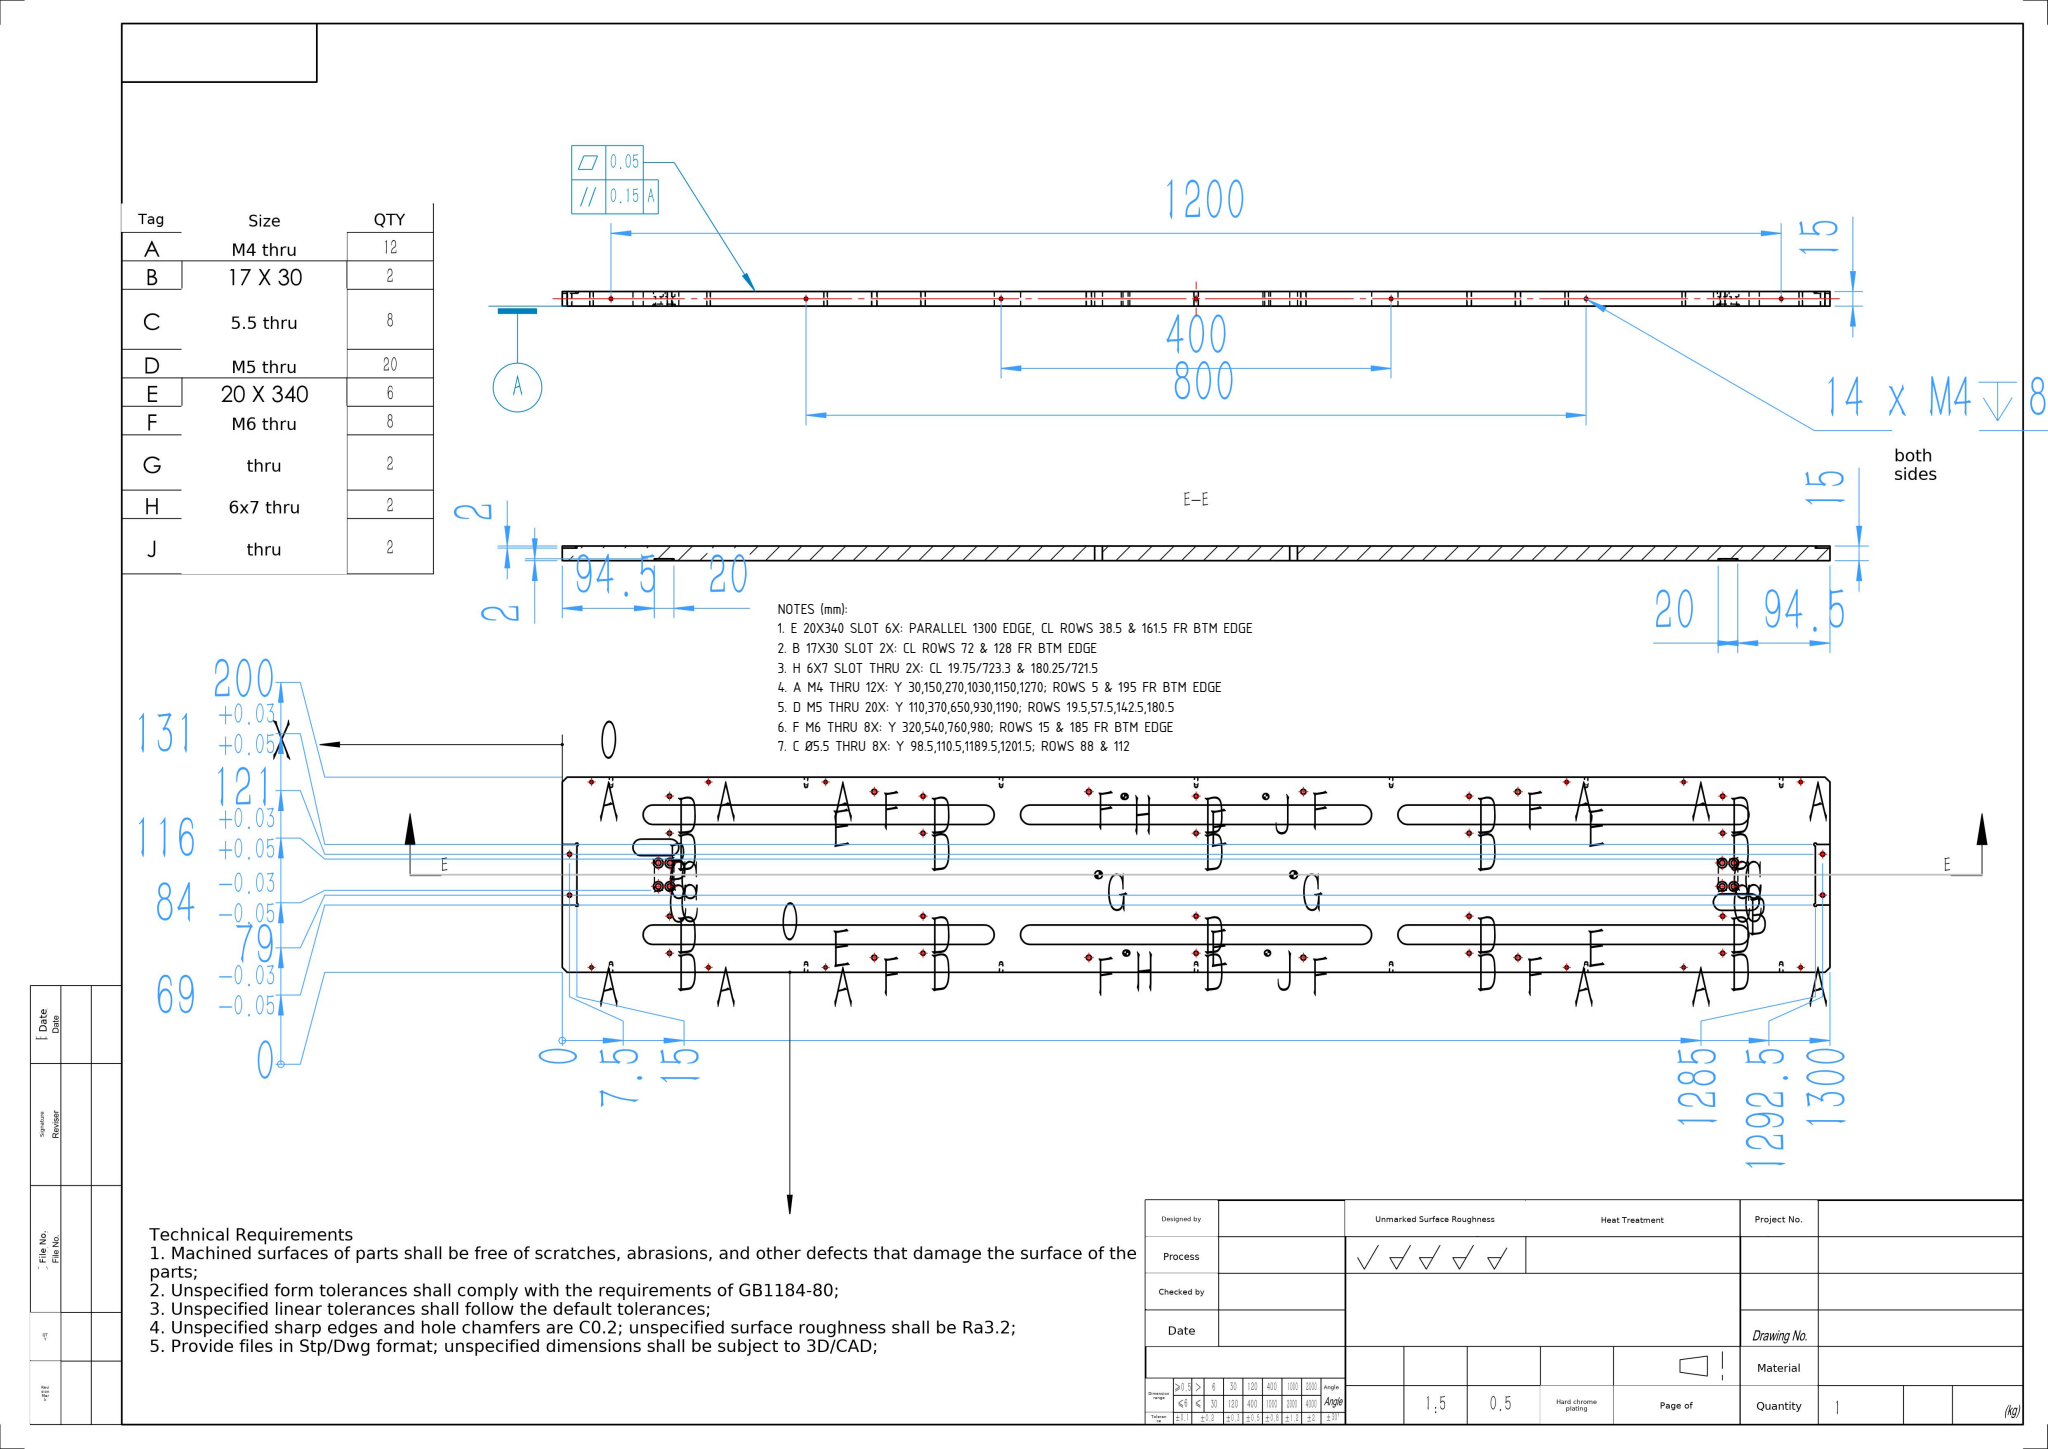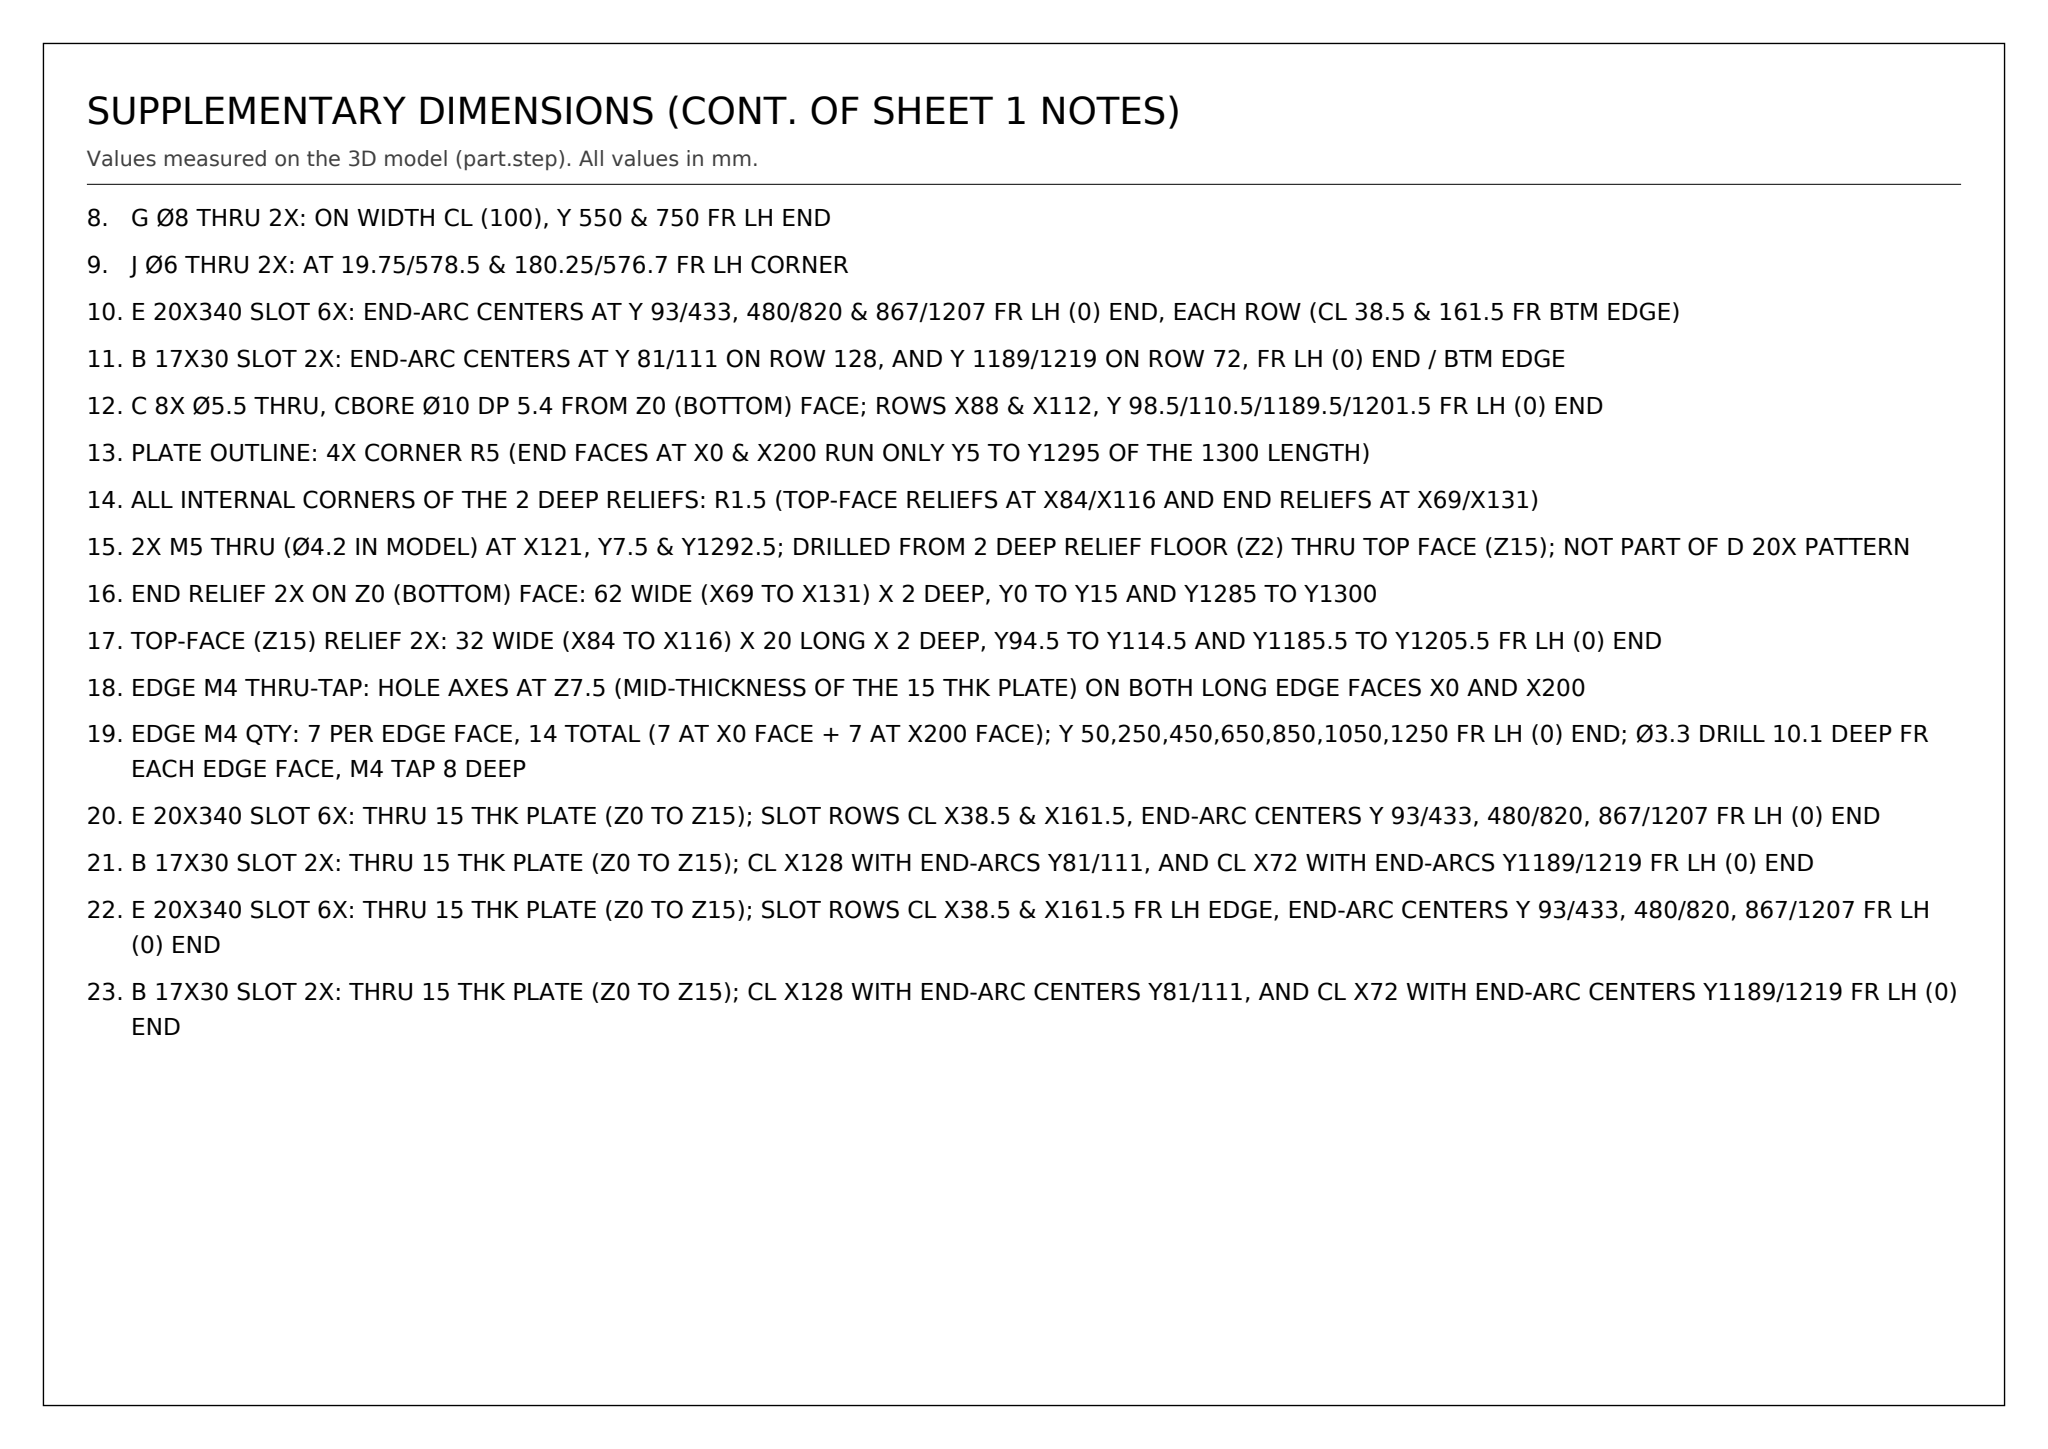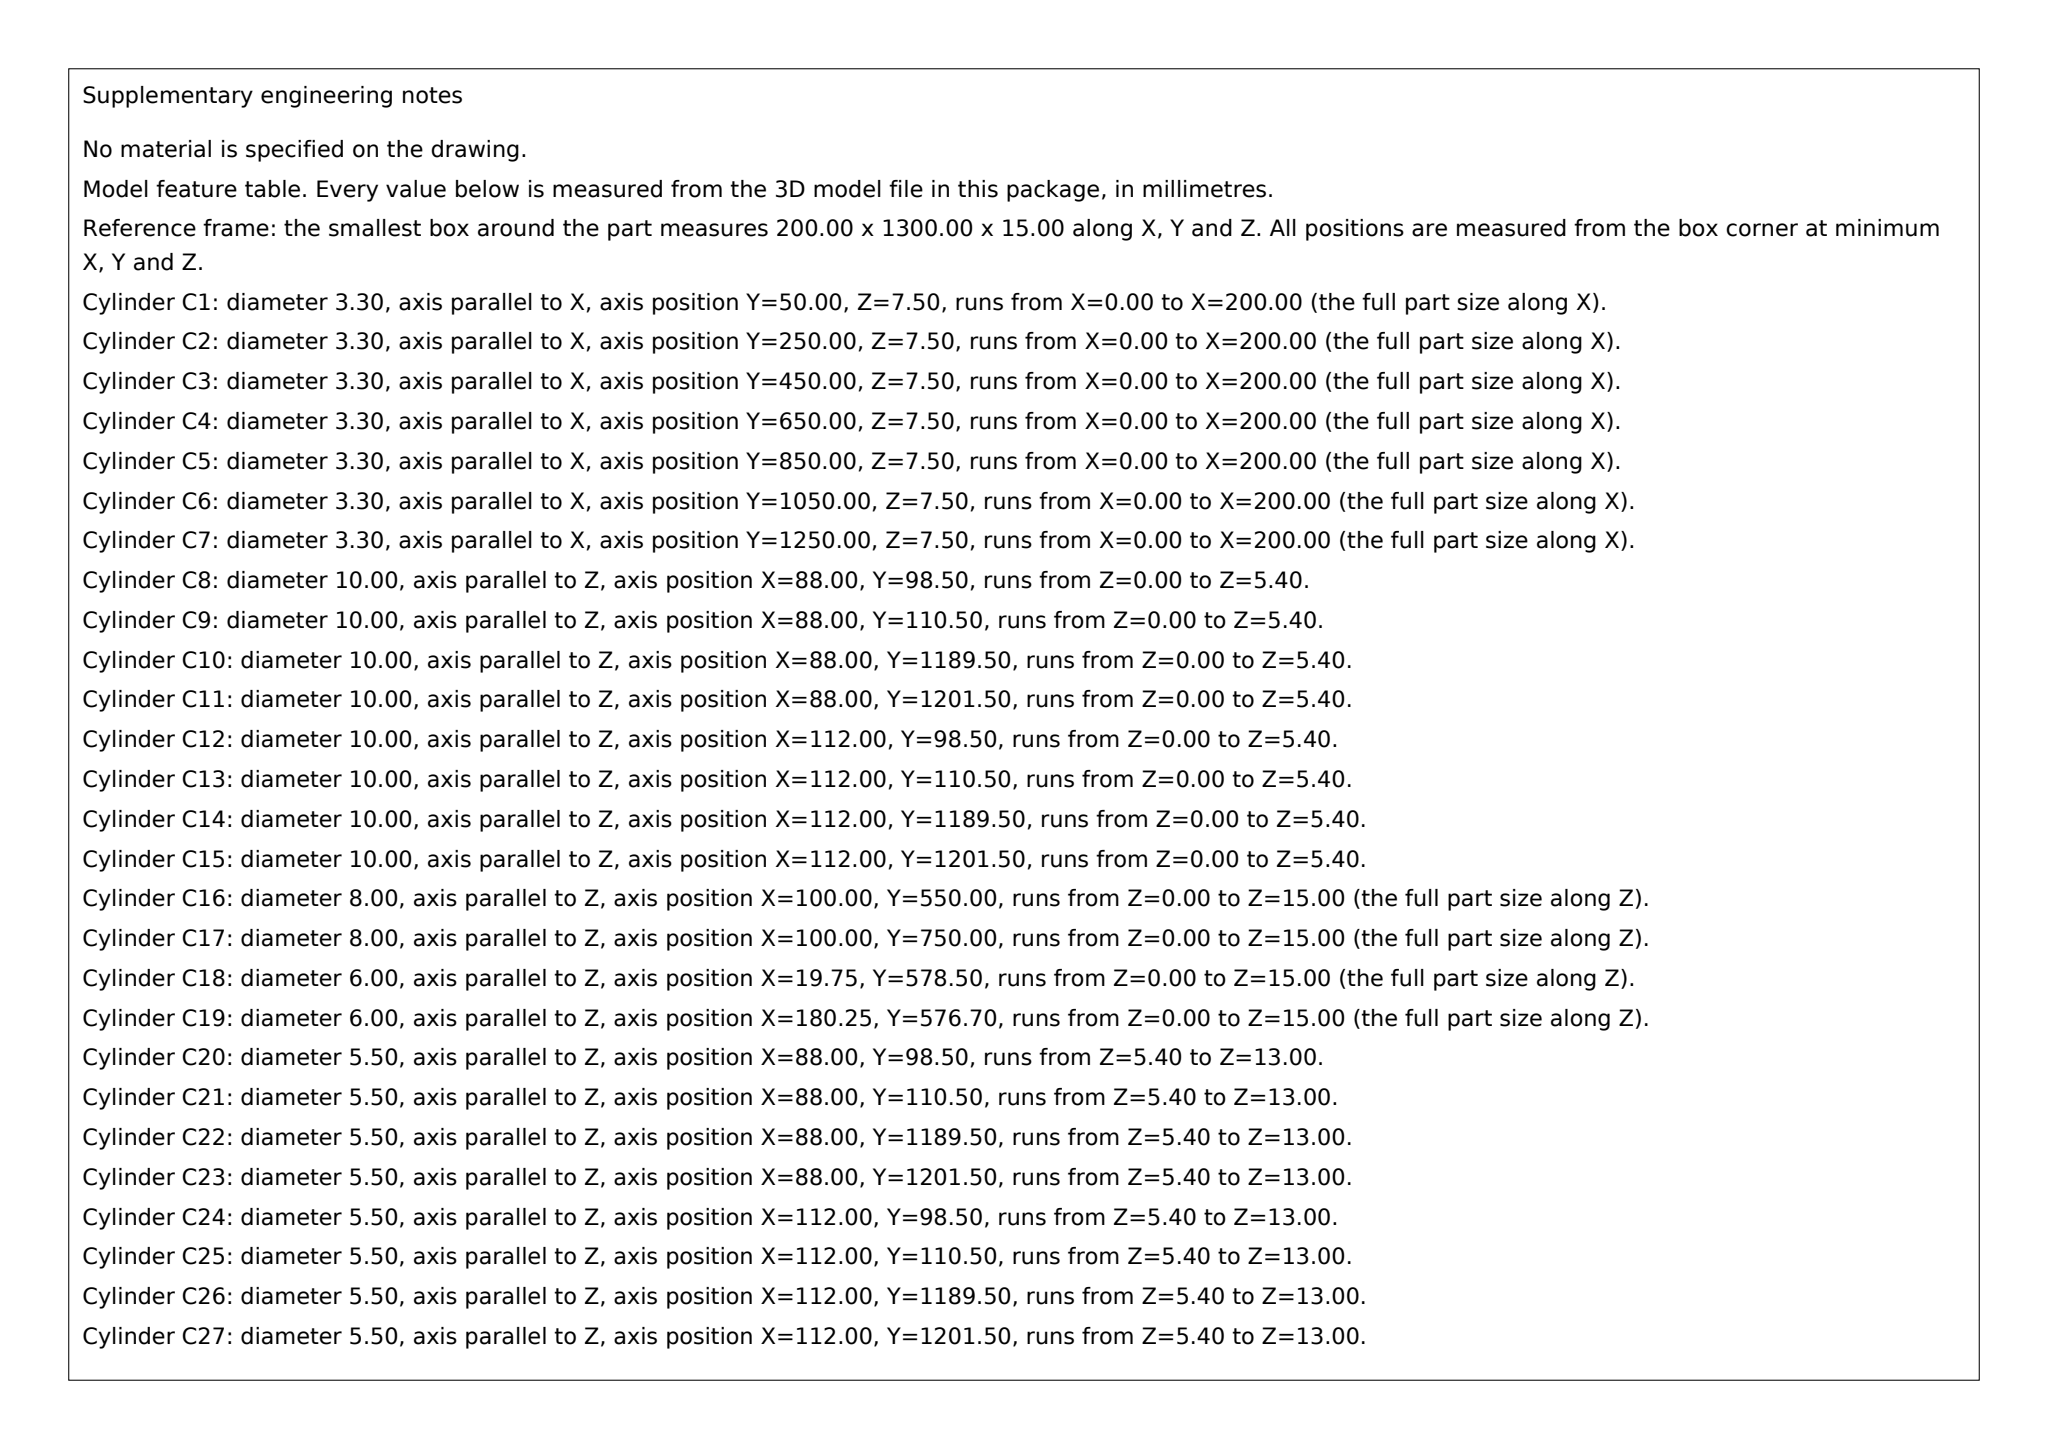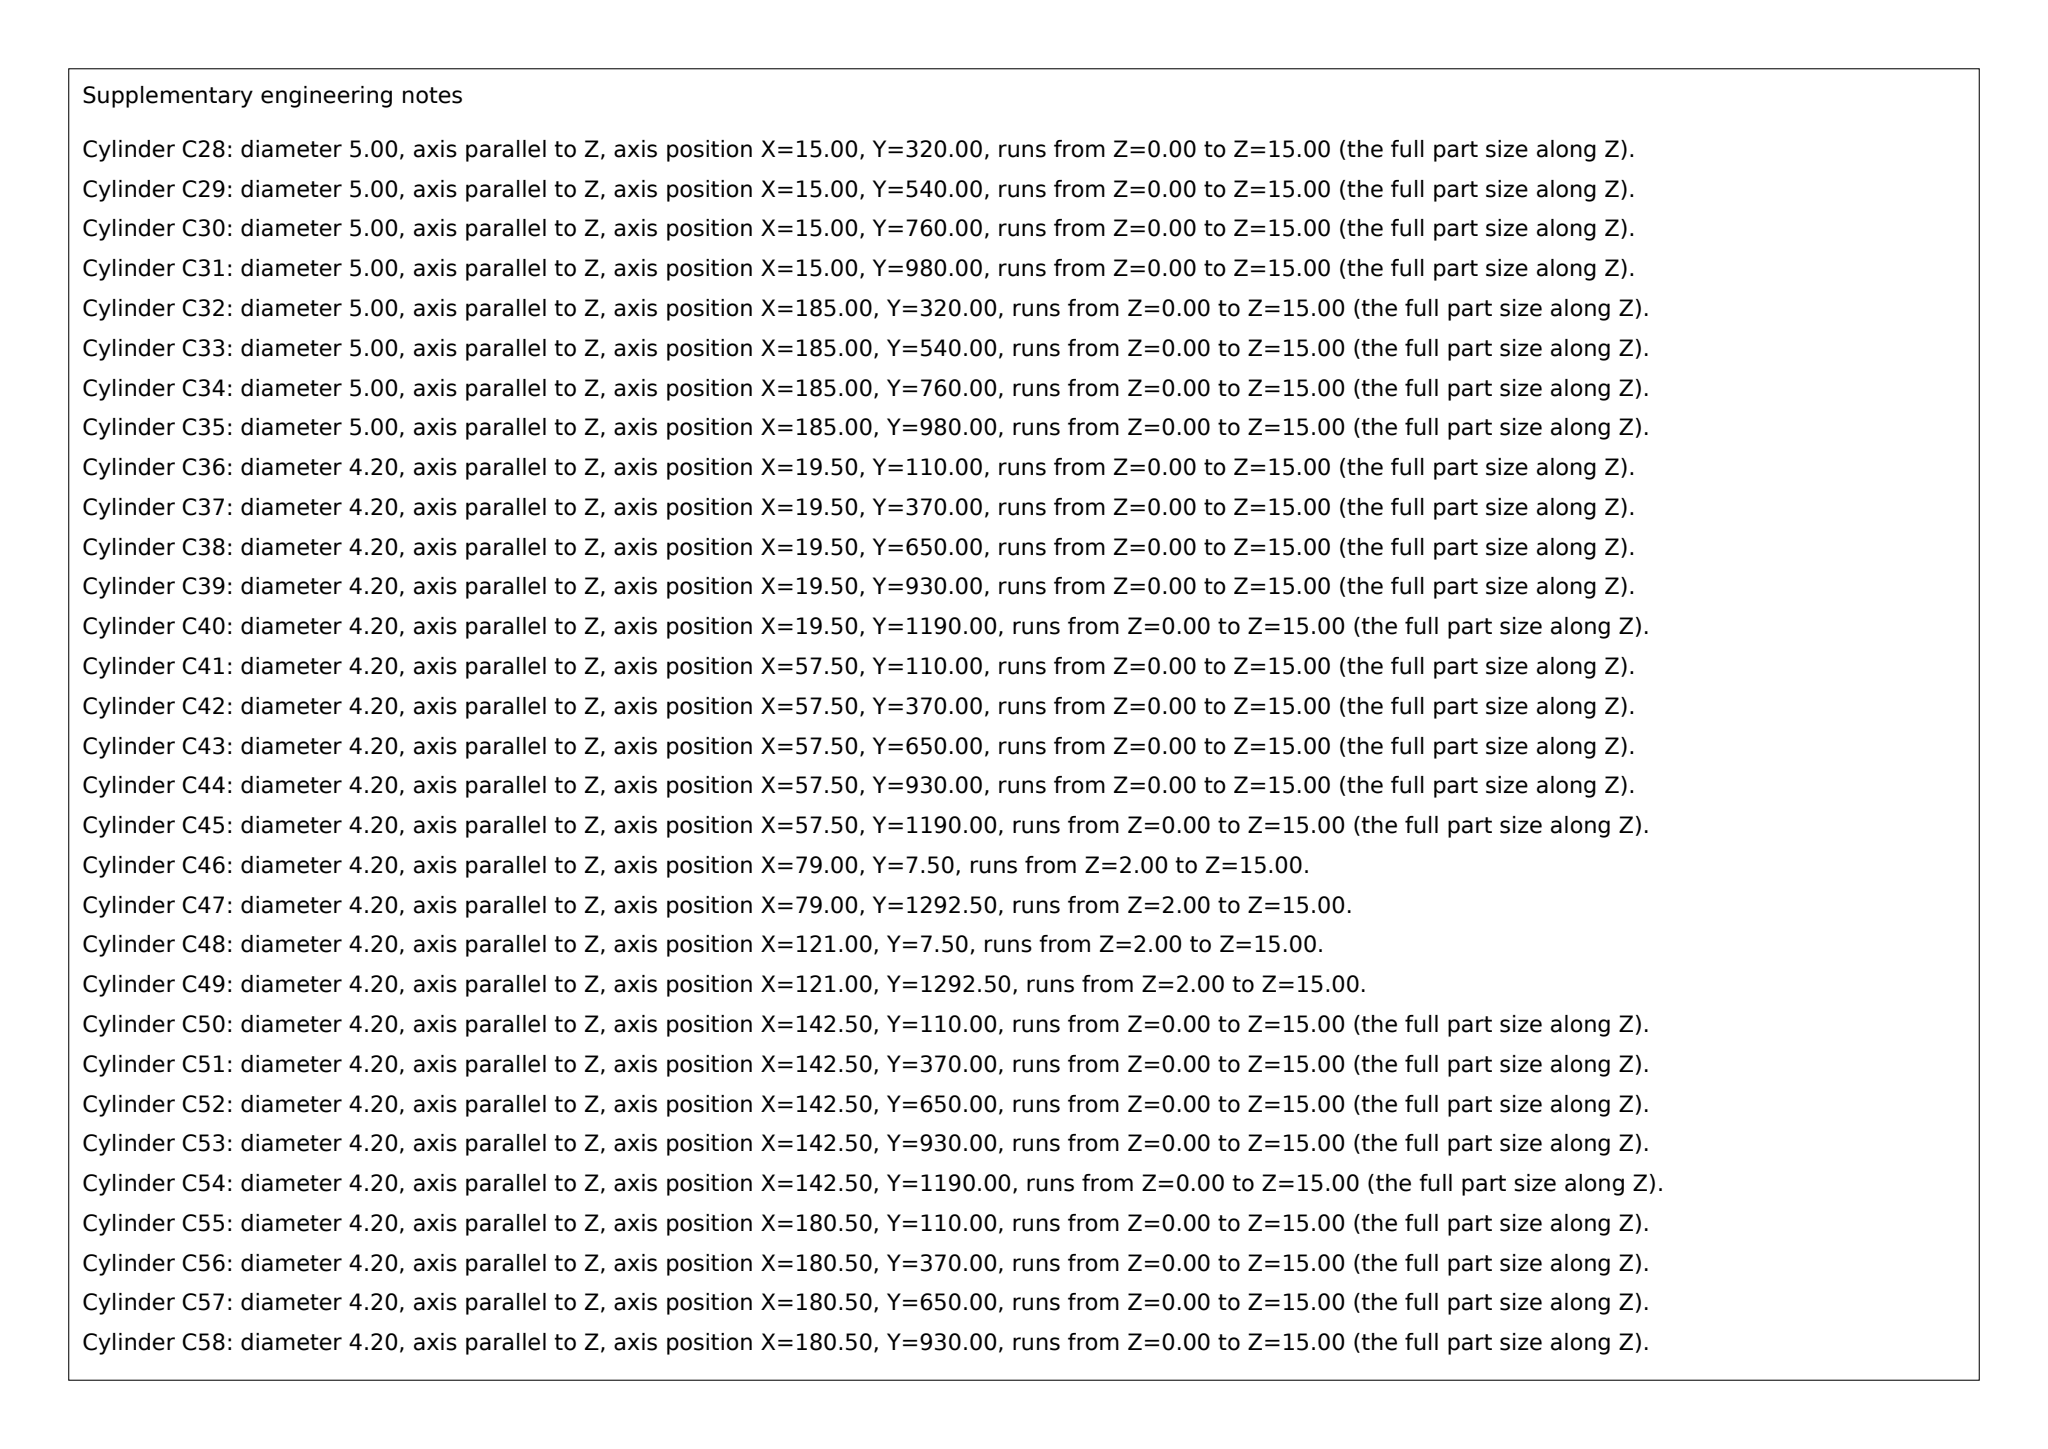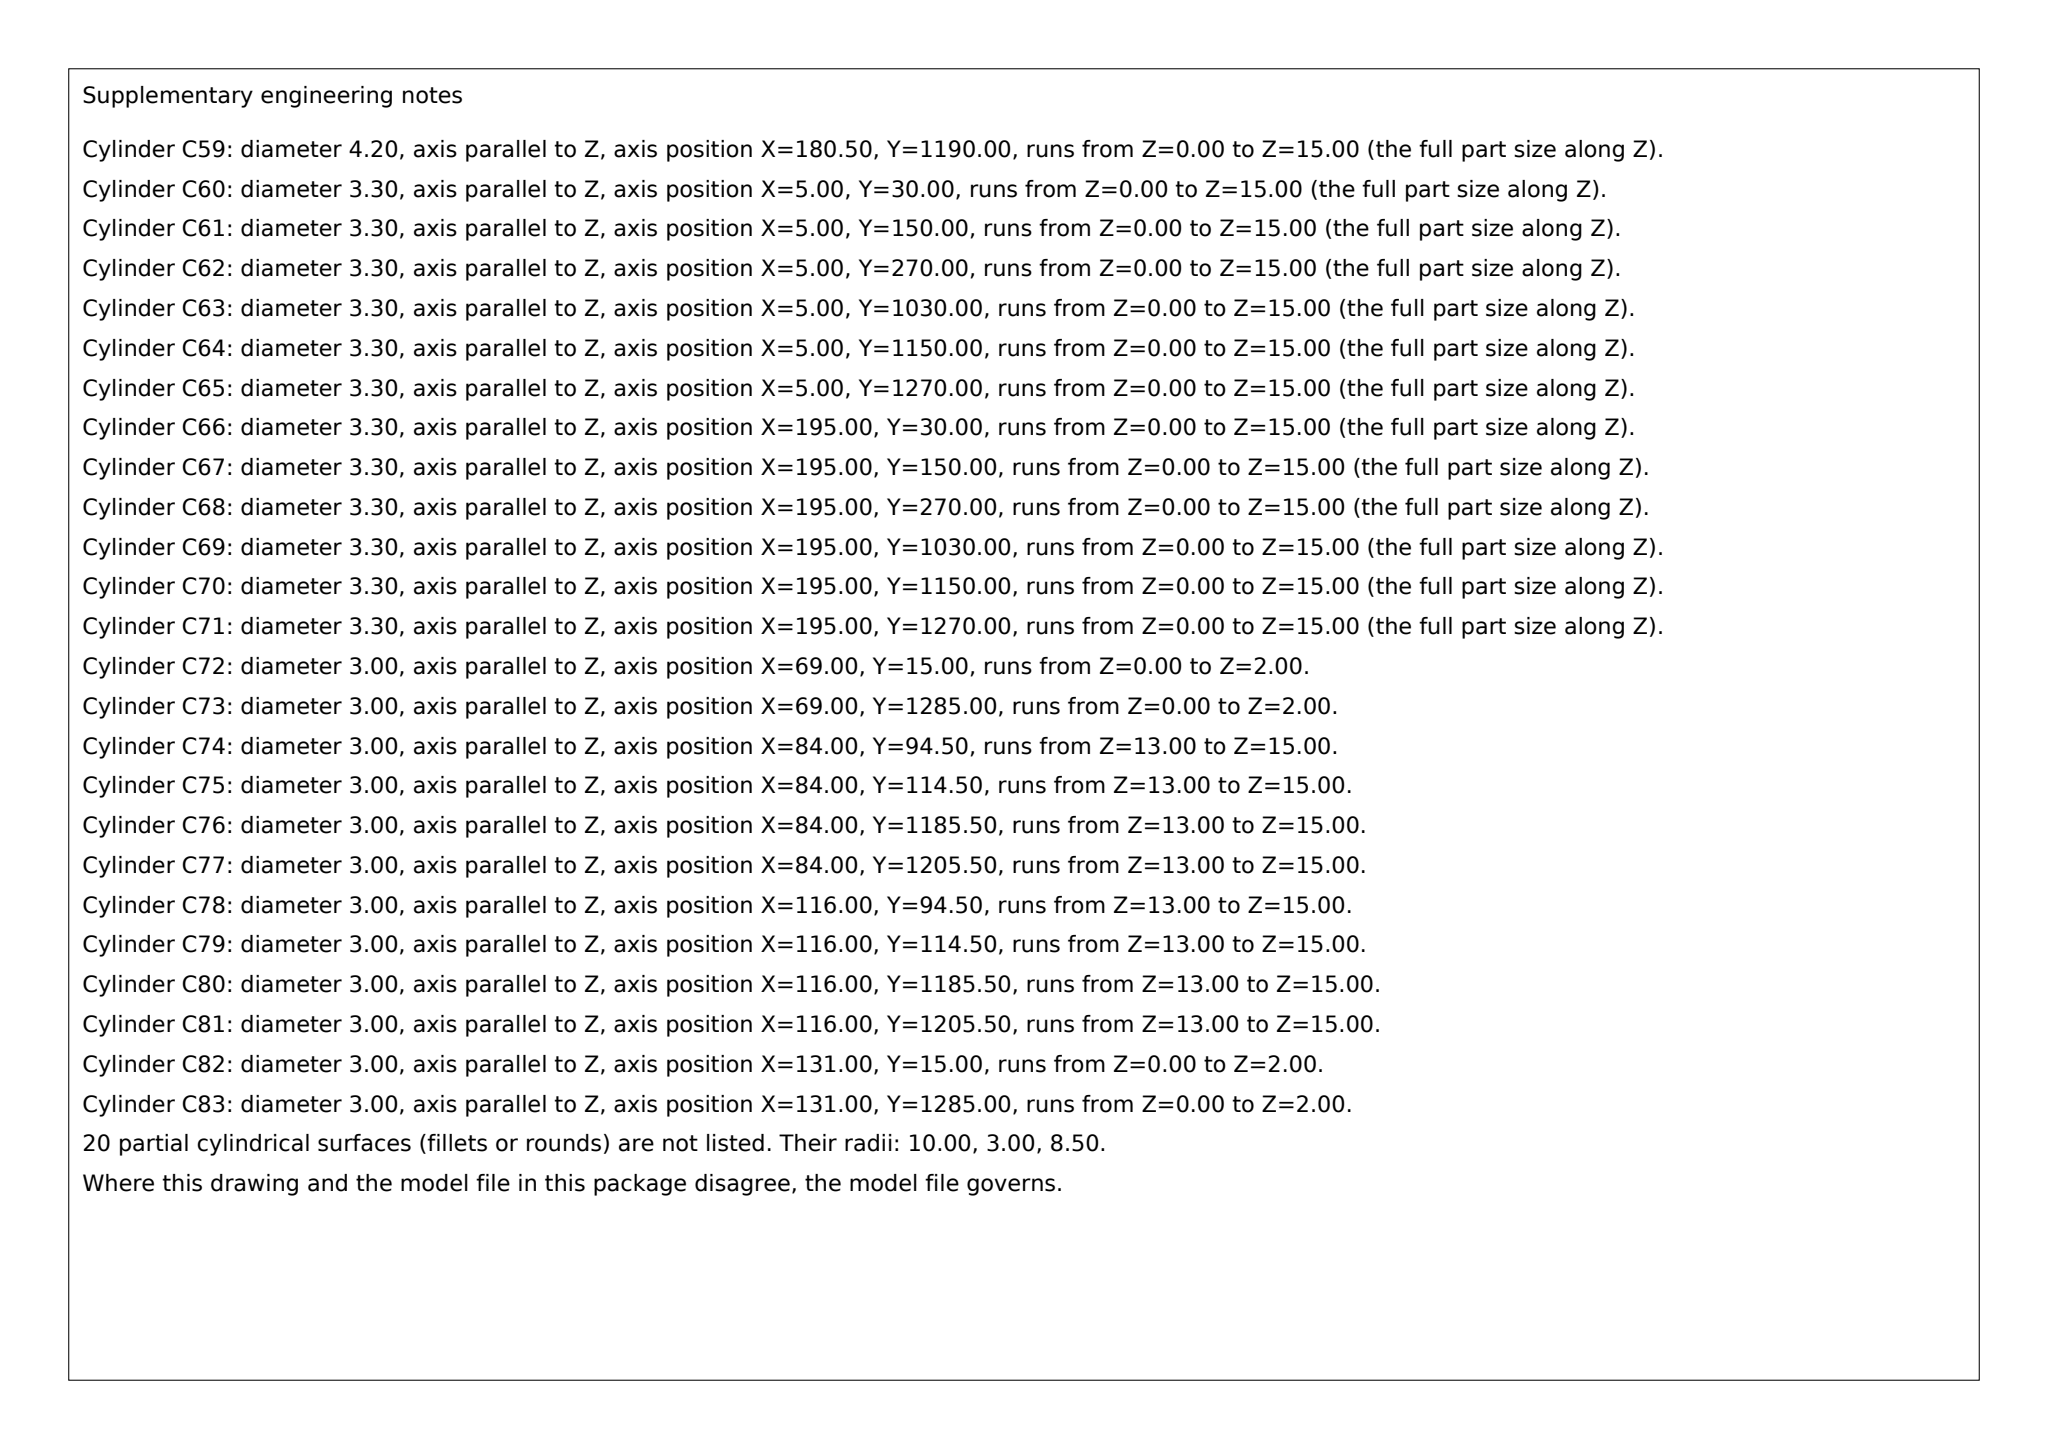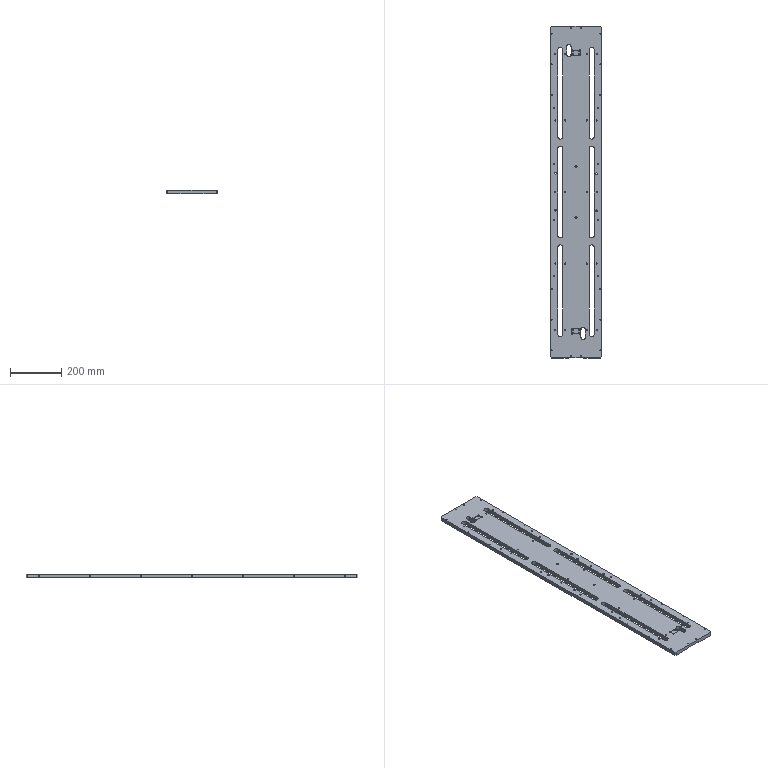Part | SolidWorks | mm | 1 solid | 278 faces | box 200 x 1300 x 15 mm | volume 3212216 mm3 | cylinder 194 | plane 56 | cone 28 | commonest cylinder face diameters 3.3 x52 4.2 x48 3 x18 10 x16 5.5 x16 5 x16 20 x12 6 x8
Drawing notes:
E 20X340 SLOT 6X: PARALLEL 1300 EDGE, CL ROWS 38.5 & 161.5 FR BTM EDGE | from the solid: x planes 28.5/48.5 (3 ea) and 151.5/171.5 (3 ea), 20 wide
B 17X30 SLOT 2X: CL ROWS 72 & 128 FR BTM EDGE | from the solid: x planes 63.5/80.5 and 119.5/136.5, 17 wide
H 6X7 SLOT THRU 2X: CL 19.75/723.3 & 180.25/721.5 | from the solid: dia 6.0 pairs 1.0 apart: (19.75,722.8/723.8) & (180.25,721.0/722.0)
A M4 THRU 12X: Y 30,150,270,1030,1150,1270; ROWS 5 & 195 FR BTM EDGE | from the solid: dia 3.3 z-holes len 15 at y=30,150,270,1030,1150,1270, x=5.0 & 195.0
D M5 THRU 20X: Y 110,370,650,930,1190; ROWS 19.5,57.5,142.5,180.5 | from the solid: dia 4.2 z-holes len 15 at y=110,370,650,930,1190; x=19.5,57.5,142.5,180.5
F M6 THRU 8X: Y 320,540,760,980; ROWS 15 & 185 FR BTM EDGE | from the solid: dia 5.0 z-holes len 15 at x=15 & 185, y=320,540,760,980
C Ø5.5 THRU 8X: Y 98.5,110.5,1189.5,1201.5; ROWS 88 & 112 | from the solid: dia 5.5 z-holes at x=88 & 112, y=98.5,110.5,1189.5,1201.5
G Ø8 THRU 2X: ON WIDTH CL (100), Y 550 & 750 FR LH END | from the solid: cyl dia 8.0 axis z at x=100, y=550 & 750, len 15 (thru)
J Ø6 THRU 2X: AT 19.75/578.5 & 180.25/576.7 FR LH CORNER | from the solid: cyl dia 6.0 axis z, len 15 thru, pos (19.75,578.5) & (180.25,576.7)
E 20X340 SLOT 6X: END-ARC CENTERS AT Y 93/433, 480/820 & 867/1207 FR LH (0) END, EACH ROW (CL 38.5 & 161.5 FR BTM EDGE) | from the solid: 20.0 dia concave slot-end arcs, z axis, at [38.5 and 161.5, y = 93,433,480,820,867,1207], from z0 to z15
B 17X30 SLOT 2X: END-ARC CENTERS AT Y 81/111 ON ROW 128, AND Y 1189/1219 ON ROW 72, FR LH (0) END / BTM EDGE | from the solid: 17.0 dia concave slot-end arcs, z axis, at [128, 81] & [128, 111] and [72, 1189] & [72, 1219], from z0 to z15
C 8X Ø5.5 THRU, CBORE Ø10 DP 5.4 FROM Z0 (BOTTOM) FACE; ROWS X88 & X112, Y 98.5/110.5/1189.5/1201.5 FR LH (0) END | from the solid: hole/bore dia 10.0 axis z at (88,98.5),(88,110.5),(88,1189.5),(88,1201.5),(112,98.5),(112,110.5),(112,1189.5),(112,1201.5) from z=0.0 to z=5.4 (360°), coaxial with Ø5.5 thru holes
PLATE OUTLINE: 4X CORNER R5 (END FACES AT X0 & X200 RUN ONLY Y5 TO Y1295 OF THE 1300 LENGTH) | from the solid: axis_planes x=0.0 and x=200.0, extent y [5.0,1295.0] z [0.0,15.0] vs bbox 200 x 1300 x 15
ALL INTERNAL CORNERS OF THE 2 DEEP RELIEFS: R1.5 (TOP-FACE RELIEFS AT X84/X116 AND END RELIEFS AT X69/X131) | from the solid: concave arcs dia 3.0 axis z at (84,94.5),(84,114.5),(116,94.5),(116,114.5),(84,1185.5),(84,1205.5),(116,1185.5),(116,1205.5) z13–15, and at (69,15),(131,15),(69,1285),(131,1285) z0–2, 270°
2X M5 THRU (Ø4.2 IN MODEL) AT X121, Y7.5 & Y1292.5; DRILLED FROM 2 DEEP RELIEF FLOOR (Z2) THRU TOP FACE (Z15); NOT PART OF D 20X PATTERN | from the solid: hole/bore dia 4.2 axis z at (121,7.5) and (121,1292.5) from z=2.0 to z=15.0
END RELIEF 2X ON Z0 (BOTTOM) FACE: 62 WIDE (X69 TO X131) X 2 DEEP, Y0 TO Y15 AND Y1285 TO Y1300 | from the solid: axis_planes x=69.0 and x=131.0, extent y [0.0,13.5] and y [1286.5,1300.0], z [0.0,2.0]; dia 3.0 arcs z0–2 at (69/131, 15 & 1285)
TOP-FACE (Z15) RELIEF 2X: 32 WIDE (X84 TO X116) X 20 LONG X 2 DEEP, Y94.5 TO Y114.5 AND Y1185.5 TO Y1205.5 FR LH (0) END | from the solid: axis_planes x=116.0 extent y [96.0,113.0] and y [1187.0,1204.0], z [13.0,15.0]; dia 3.0 corner arcs z13–15 at X84 & X116, Y94.5/114.5/1185.5/1205.5
EDGE M4 THRU-TAP: HOLE AXES AT Z7.5 (MID-THICKNESS OF THE 15 THK PLATE) ON BOTH LONG EDGE FACES X0 AND X200 | from the solid: cylinders: hole/bore dia 3.3, axis x, axis_pos [y, z=7.5], from 0.0 to 10.1 and from 189.9 to 200.0; bbox_xyz z = 15.0
EDGE M4 QTY: 7 PER EDGE FACE, 14 TOTAL (7 AT X0 FACE + 7 AT X200 FACE); Y 50,250,450,650,850,1050,1250 FR LH (0) END; Ø3.3 DRILL 10.1 DEEP FR EACH EDGE FACE, M4 TAP 8 DEEP | from the solid: cylinders: 14 off hole/bore dia 3.3 axis x at y = 50,250,450,650,850,1050,1250; seven from 0.0 to 10.1 (X0 face) and seven from 189.9 to 200.0 (X200 face)
E 20X340 SLOT 6X: THRU 15 THK PLATE (Z0 TO Z15); SLOT ROWS CL X38.5 & X161.5, END-ARC CENTERS Y 93/433, 480/820, 867/1207 FR LH (0) END | from the solid: Ø20 z-axis slot-end arcs at [38.5/161.5, Y93,433,480,820,867,1207] run from z=0.0 to z=15.0; slot side planes x=28.5/48.5/151.5/171.5 extent z [0.0,15.0] on 15 thk bbox
B 17X30 SLOT 2X: THRU 15 THK PLATE (Z0 TO Z15); CL X128 WITH END-ARCS Y81/111, AND CL X72 WITH END-ARCS Y1189/1219 FR LH (0) END | from the solid: Ø17 z-axis slot-end arcs at [128, Y81/111] and [72, Y1189/1219] run from z=0.0 to z=15.0; slot side planes x=119.5/136.5 and x=63.5/80.5 extent z [0.0,15.0]
E 20X340 SLOT 6X: THRU 15 THK PLATE (Z0 TO Z15); SLOT ROWS CL X38.5 & X161.5 FR LH EDGE, END-ARC CENTERS Y 93/433, 480/820, 867/1207 FR LH (0) END | from the solid: 20.0 dia 180-deg slot-end arcs, axis z at (38.5/161.5, Y 93,433,480,820,867,1207), from z 0.0 to 15.0; slot side planes x=28.5/48.5 and x=151.5/171.5 with z extent [0,15]
B 17X30 SLOT 2X: THRU 15 THK PLATE (Z0 TO Z15); CL X128 WITH END-ARC CENTERS Y81/111, AND CL X72 WITH END-ARC CENTERS Y1189/1219 FR LH (0) END | from the solid: 17.0 dia 180-deg slot-end arcs, axis z at (128, Y81/111) and (72, Y1189/1219), from z 0.0 to 15.0; slot side planes x=119.5/136.5 and x=63.5/80.5 with z extent [0,15]